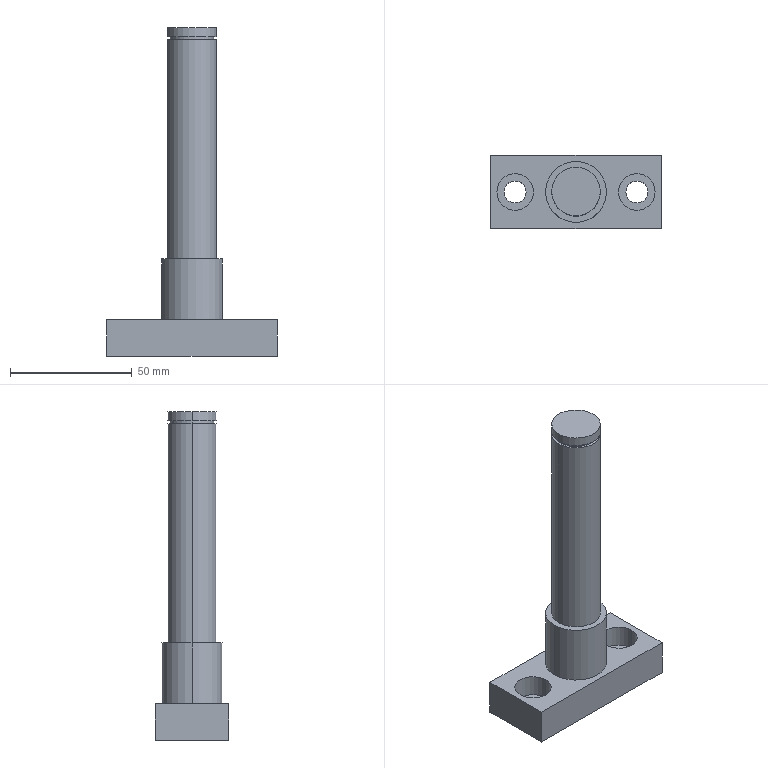Component | SolidWorks | -SmallRollerAssembly-1_-SmallPulleyBearingHousing-1 | 1 solid | 28 faces | box 70 x 30 x 135 mm | volume 69601 mm3 | cylinder 16 | plane 12 | commonest cylinder face diameters 15 x4 9 x4 20 x4 18 x2 25 x2
build123d program:
from build123d import *

# Parameters (mm, degrees)
SKETCH1_W                                           = 70
SKETCH1_H                                           = 30
BOSS_EXTRUDE1_DEPTH                                 = 15
SKETCH2_R                                           = 12.5
BOSS_EXTRUDE2_DEPTH                                 = 25
SKETCH3_R                                           = 10
BOSS_EXTRUDE3_DEPTH                                 = 95
SKETCH4_R                                           = 10
SKETCH4_R_2                                         = 9
CUT_EXTRUDE1_DEPTH                                  = 1.2
CYLINDRICAL_COUNTERSUNK_HOLE_FOR_M8_HEX_D           = 9
CYLINDRICAL_COUNTERSUNK_HOLE_FOR_M8_HEX_CBORE_D     = 15
CYLINDRICAL_COUNTERSUNK_HOLE_FOR_M8_HEX_CBORE_DEPTH = 9


with BuildPart() as part:
    # Sketch1 → Boss-Extrude1 (new body)
    with BuildSketch(Plane.XY):
        Rectangle(SKETCH1_W, SKETCH1_H)
    extrude(amount=BOSS_EXTRUDE1_DEPTH)

    # Sketch2 → Boss-Extrude2 (add)
    with BuildSketch(Plane.XY.offset(15)):
        Circle(SKETCH2_R)
    extrude(amount=BOSS_EXTRUDE2_DEPTH)

    # Sketch3 → Boss-Extrude3 (add)
    with BuildSketch(Plane.XY.offset(40)):
        Circle(SKETCH3_R)
    extrude(amount=BOSS_EXTRUDE3_DEPTH)

    # Sketch4 → Cut-Extrude1 (cut)
    with BuildSketch(Plane.XY.offset(130)):
        Circle(SKETCH4_R)
        Circle(SKETCH4_R_2, mode=Mode.SUBTRACT)
    extrude(amount=CUT_EXTRUDE1_DEPTH, mode=Mode.SUBTRACT)

    # Cylindrical Countersunk Hole for M8 Hex (through all)
    with Locations(Plane(origin=(0, 0, 15), x_dir=(-1, 0, 0), z_dir=(0, 0, 1))):
        with Locations((-25, 0), (25, 0)):
            CounterBoreHole(CYLINDRICAL_COUNTERSUNK_HOLE_FOR_M8_HEX_D / 2, CYLINDRICAL_COUNTERSUNK_HOLE_FOR_M8_HEX_CBORE_D / 2, CYLINDRICAL_COUNTERSUNK_HOLE_FOR_M8_HEX_CBORE_DEPTH)


solid = part.part

# Placed as in the assembly
solid = solid.moved(Location((-45, 1121, 5), (0, 0, 0)))
STEP:
#1=COLOUR_RGB('',0.7922,0.8196,0.9333);
#2=FILL_AREA_STYLE_COLOUR('',#1);
#3=FILL_AREA_STYLE('',(#2));
#4=SURFACE_STYLE_FILL_AREA(#3);
#5=SURFACE_SIDE_STYLE('',(#4));
#6=SURFACE_STYLE_USAGE(.BOTH.,#5);
#7=PRESENTATION_STYLE_ASSIGNMENT((#6));
#8=CARTESIAN_POINT('',(-1.083,44.134,0.4331));
#9=VERTEX_POINT('',#8);
#10=CARTESIAN_POINT('',(-0.4921,44.134,0.4331));
#11=VERTEX_POINT('',#10);
#12=CARTESIAN_POINT('',(-0.7874,44.134,0.4331));
#13=DIRECTION('',(0.,0.,1.));
#14=DIRECTION('',(1.,0.,0.));
#15=AXIS2_PLACEMENT_3D('',#12,#13,#14);
#16=CIRCLE('',#15,0.2953);
#17=EDGE_CURVE('',#9,#11,#16,.T.);
#18=ORIENTED_EDGE('',*,*,#17,.F.);
#19=CARTESIAN_POINT('',(-1.083,44.134,0.7874));
#20=VERTEX_POINT('',#19);
#21=CARTESIAN_POINT('',(-1.083,44.134,0.7874));
#22=DIRECTION('',(0.,0.,1.));
#23=VECTOR('',#22,39.37);
#24=LINE('',#21,#23);
#25=EDGE_CURVE('',#9,#20,#24,.T.);
#26=ORIENTED_EDGE('',*,*,#25,.T.);
#27=CARTESIAN_POINT('',(-0.4921,44.134,0.7874));
#28=VERTEX_POINT('',#27);
#29=CARTESIAN_POINT('',(-0.7874,44.134,0.7874));
#30=DIRECTION('',(0.,0.,1.));
#31=DIRECTION('',(1.,0.,0.));
#32=AXIS2_PLACEMENT_3D('',#29,#30,#31);
#33=CIRCLE('',#32,0.2953);
#34=EDGE_CURVE('',#20,#28,#33,.T.);
#35=ORIENTED_EDGE('',*,*,#34,.T.);
#36=CARTESIAN_POINT('',(-0.4921,44.134,0.7874));
#37=DIRECTION('',(0.,0.,1.));
#38=VECTOR('',#37,39.37);
#39=LINE('',#36,#38);
#40=EDGE_CURVE('',#11,#28,#39,.T.);
#41=ORIENTED_EDGE('',*,*,#40,.F.);
#42=EDGE_LOOP('',(#18,#26,#35,#41));
#43=FACE_OUTER_BOUND('',#42,.T.);
#44=CARTESIAN_POINT('',(-0.7874,44.134,0.7874));
#45=DIRECTION('',(0.,0.,1.));
#46=DIRECTION('',(1.,0.,0.));
#47=AXIS2_PLACEMENT_3D('',#44,#45,#46);
#48=CYLINDRICAL_SURFACE('',#47,0.2953);
#49=ADVANCED_FACE('',(#43),#48,.F.);
#50=CARTESIAN_POINT('',(-0.9646,44.134,0.1969));
#51=VERTEX_POINT('',#50);
#52=CARTESIAN_POINT('',(-0.6102,44.134,0.1969));
#53=VERTEX_POINT('',#52);
#54=CARTESIAN_POINT('',(-0.7874,44.134,0.1969));
#55=DIRECTION('',(0.,0.,1.));
#56=DIRECTION('',(1.,0.,0.));
#57=AXIS2_PLACEMENT_3D('',#54,#55,#56);
#58=CIRCLE('',#57,0.1772);
#59=EDGE_CURVE('',#51,#53,#58,.T.);
#60=ORIENTED_EDGE('',*,*,#59,.F.);
#61=CARTESIAN_POINT('',(-0.9646,44.134,0.4331));
#62=VERTEX_POINT('',#61);
#63=CARTESIAN_POINT('',(-0.9646,44.134,0.7874));
#64=DIRECTION('',(0.,0.,1.));
#65=VECTOR('',#64,39.37);
#66=LINE('',#63,#65);
#67=EDGE_CURVE('',#51,#62,#66,.T.);
#68=ORIENTED_EDGE('',*,*,#67,.T.);
#69=CARTESIAN_POINT('',(-0.6102,44.134,0.4331));
#70=VERTEX_POINT('',#69);
#71=CARTESIAN_POINT('',(-0.7874,44.134,0.4331));
#72=DIRECTION('',(0.,0.,1.));
#73=DIRECTION('',(1.,0.,0.));
#74=AXIS2_PLACEMENT_3D('',#71,#72,#73);
#75=CIRCLE('',#74,0.1772);
#76=EDGE_CURVE('',#62,#70,#75,.T.);
#77=ORIENTED_EDGE('',*,*,#76,.T.);
#78=CARTESIAN_POINT('',(-0.6102,44.134,0.7874));
#79=DIRECTION('',(0.,0.,1.));
#80=VECTOR('',#79,39.37);
#81=LINE('',#78,#80);
#82=EDGE_CURVE('',#53,#70,#81,.T.);
#83=ORIENTED_EDGE('',*,*,#82,.F.);
#84=EDGE_LOOP('',(#60,#68,#77,#83));
#85=FACE_OUTER_BOUND('',#84,.T.);
#86=CARTESIAN_POINT('',(-0.7874,44.134,0.7874));
#87=DIRECTION('',(0.,0.,1.));
#88=DIRECTION('',(1.,0.,0.));
#89=AXIS2_PLACEMENT_3D('',#86,#87,#88);
#90=CYLINDRICAL_SURFACE('',#89,0.1772);
#91=ADVANCED_FACE('',(#85),#90,.F.);
#92=CARTESIAN_POINT('',(-3.051,44.134,0.4331));
#93=VERTEX_POINT('',#92);
#94=CARTESIAN_POINT('',(-2.461,44.134,0.4331));
#95=VERTEX_POINT('',#94);
#96=CARTESIAN_POINT('',(-2.756,44.134,0.4331));
#97=DIRECTION('',(0.,0.,1.));
#98=DIRECTION('',(1.,0.,0.));
#99=AXIS2_PLACEMENT_3D('',#96,#97,#98);
#100=CIRCLE('',#99,0.2953);
#101=EDGE_CURVE('',#93,#95,#100,.T.);
#102=ORIENTED_EDGE('',*,*,#101,.F.);
#103=CARTESIAN_POINT('',(-3.051,44.134,0.7874));
#104=VERTEX_POINT('',#103);
#105=CARTESIAN_POINT('',(-3.051,44.134,0.7874));
#106=DIRECTION('',(0.,0.,1.));
#107=VECTOR('',#106,39.37);
#108=LINE('',#105,#107);
#109=EDGE_CURVE('',#93,#104,#108,.T.);
#110=ORIENTED_EDGE('',*,*,#109,.T.);
#111=CARTESIAN_POINT('',(-2.461,44.134,0.7874));
#112=VERTEX_POINT('',#111);
#113=CARTESIAN_POINT('',(-2.756,44.134,0.7874));
#114=DIRECTION('',(0.,0.,1.));
#115=DIRECTION('',(1.,0.,0.));
#116=AXIS2_PLACEMENT_3D('',#113,#114,#115);
#117=CIRCLE('',#116,0.2953);
#118=EDGE_CURVE('',#104,#112,#117,.T.);
#119=ORIENTED_EDGE('',*,*,#118,.T.);
#120=CARTESIAN_POINT('',(-2.461,44.134,0.7874));
#121=DIRECTION('',(0.,0.,1.));
#122=VECTOR('',#121,39.37);
#123=LINE('',#120,#122);
#124=EDGE_CURVE('',#95,#112,#123,.T.);
#125=ORIENTED_EDGE('',*,*,#124,.F.);
#126=EDGE_LOOP('',(#102,#110,#119,#125));
#127=FACE_OUTER_BOUND('',#126,.T.);
#128=CARTESIAN_POINT('',(-2.756,44.134,0.7874));
#129=DIRECTION('',(0.,0.,1.));
#130=DIRECTION('',(1.,0.,0.));
#131=AXIS2_PLACEMENT_3D('',#128,#129,#130);
#132=CYLINDRICAL_SURFACE('',#131,0.2953);
#133=ADVANCED_FACE('',(#127),#132,.F.);
#134=CARTESIAN_POINT('',(-2.933,44.134,0.1969));
#135=VERTEX_POINT('',#134);
#136=CARTESIAN_POINT('',(-2.579,44.134,0.1969));
#137=VERTEX_POINT('',#136);
#138=CARTESIAN_POINT('',(-2.756,44.134,0.1969));
#139=DIRECTION('',(0.,0.,1.));
#140=DIRECTION('',(1.,0.,0.));
#141=AXIS2_PLACEMENT_3D('',#138,#139,#140);
#142=CIRCLE('',#141,0.1772);
#143=EDGE_CURVE('',#135,#137,#142,.T.);
#144=ORIENTED_EDGE('',*,*,#143,.F.);
#145=CARTESIAN_POINT('',(-2.933,44.134,0.4331));
#146=VERTEX_POINT('',#145);
#147=CARTESIAN_POINT('',(-2.933,44.134,0.7874));
#148=DIRECTION('',(0.,0.,1.));
#149=VECTOR('',#148,39.37);
#150=LINE('',#147,#149);
#151=EDGE_CURVE('',#135,#146,#150,.T.);
#152=ORIENTED_EDGE('',*,*,#151,.T.);
#153=CARTESIAN_POINT('',(-2.579,44.134,0.4331));
#154=VERTEX_POINT('',#153);
#155=CARTESIAN_POINT('',(-2.756,44.134,0.4331));
#156=DIRECTION('',(0.,0.,1.));
#157=DIRECTION('',(1.,0.,0.));
#158=AXIS2_PLACEMENT_3D('',#155,#156,#157);
#159=CIRCLE('',#158,0.1772);
#160=EDGE_CURVE('',#146,#154,#159,.T.);
#161=ORIENTED_EDGE('',*,*,#160,.T.);
#162=CARTESIAN_POINT('',(-2.579,44.134,0.7874));
#163=DIRECTION('',(0.,0.,1.));
#164=VECTOR('',#163,39.37);
#165=LINE('',#162,#164);
#166=EDGE_CURVE('',#137,#154,#165,.T.);
#167=ORIENTED_EDGE('',*,*,#166,.F.);
#168=EDGE_LOOP('',(#144,#152,#161,#167));
#169=FACE_OUTER_BOUND('',#168,.T.);
#170=CARTESIAN_POINT('',(-2.756,44.134,0.7874));
#171=DIRECTION('',(0.,0.,1.));
#172=DIRECTION('',(1.,0.,0.));
#173=AXIS2_PLACEMENT_3D('',#170,#171,#172);
#174=CYLINDRICAL_SURFACE('',#173,0.1772);
#175=ADVANCED_FACE('',(#169),#174,.F.);
#176=CARTESIAN_POINT('',(-1.378,44.134,5.512));
#177=VERTEX_POINT('',#176);
#178=CARTESIAN_POINT('',(-2.165,44.134,5.512));
#179=VERTEX_POINT('',#178);
#180=CARTESIAN_POINT('',(-1.772,44.134,5.512));
#181=DIRECTION('',(0.,0.,1.));
#182=DIRECTION('',(1.,0.,0.));
#183=AXIS2_PLACEMENT_3D('',#180,#181,#182);
#184=CIRCLE('',#183,0.3937);
#185=EDGE_CURVE('',#177,#179,#184,.T.);
#186=ORIENTED_EDGE('',*,*,#185,.F.);
#187=CARTESIAN_POINT('',(-1.378,44.134,5.362));
#188=VERTEX_POINT('',#187);
#189=CARTESIAN_POINT('',(-1.378,44.134,5.512));
#190=DIRECTION('',(0.,0.,-1.));
#191=VECTOR('',#190,39.37);
#192=LINE('',#189,#191);
#193=EDGE_CURVE('',#177,#188,#192,.T.);
#194=ORIENTED_EDGE('',*,*,#193,.T.);
#195=CARTESIAN_POINT('',(-2.165,44.134,5.362));
#196=VERTEX_POINT('',#195);
#197=CARTESIAN_POINT('',(-1.772,44.134,5.362));
#198=DIRECTION('',(0.,0.,1.));
#199=DIRECTION('',(1.,0.,0.));
#200=AXIS2_PLACEMENT_3D('',#197,#198,#199);
#201=CIRCLE('',#200,0.3937);
#202=EDGE_CURVE('',#188,#196,#201,.T.);
#203=ORIENTED_EDGE('',*,*,#202,.T.);
#204=CARTESIAN_POINT('',(-2.165,44.134,5.512));
#205=DIRECTION('',(0.,0.,-1.));
#206=VECTOR('',#205,39.37);
#207=LINE('',#204,#206);
#208=EDGE_CURVE('',#179,#196,#207,.T.);
#209=ORIENTED_EDGE('',*,*,#208,.F.);
#210=EDGE_LOOP('',(#186,#194,#203,#209));
#211=FACE_OUTER_BOUND('',#210,.T.);
#212=CARTESIAN_POINT('',(-1.772,44.134,5.512));
#213=DIRECTION('',(0.,0.,-1.));
#214=DIRECTION('',(-1.,0.,0.));
#215=AXIS2_PLACEMENT_3D('',#212,#213,#214);
#216=CYLINDRICAL_SURFACE('',#215,0.3937);
#217=ADVANCED_FACE('',(#211),#216,.T.);
#218=CARTESIAN_POINT('',(-1.417,44.134,5.362));
#219=VERTEX_POINT('',#218);
#220=CARTESIAN_POINT('',(-2.126,44.134,5.362));
#221=VERTEX_POINT('',#220);
#222=CARTESIAN_POINT('',(-1.772,44.134,5.362));
#223=DIRECTION('',(0.,0.,1.));
#224=DIRECTION('',(1.,0.,0.));
#225=AXIS2_PLACEMENT_3D('',#222,#223,#224);
#226=CIRCLE('',#225,0.3543);
#227=EDGE_CURVE('',#219,#221,#226,.T.);
#228=ORIENTED_EDGE('',*,*,#227,.F.);
#229=CARTESIAN_POINT('',(-1.417,44.134,5.315));
#230=VERTEX_POINT('',#229);
#231=CARTESIAN_POINT('',(-1.417,44.134,5.362));
#232=DIRECTION('',(0.,0.,-1.));
#233=VECTOR('',#232,39.37);
#234=LINE('',#231,#233);
#235=EDGE_CURVE('',#219,#230,#234,.T.);
#236=ORIENTED_EDGE('',*,*,#235,.T.);
#237=CARTESIAN_POINT('',(-2.126,44.134,5.315));
#238=VERTEX_POINT('',#237);
#239=CARTESIAN_POINT('',(-1.772,44.134,5.315));
#240=DIRECTION('',(0.,0.,1.));
#241=DIRECTION('',(1.,0.,0.));
#242=AXIS2_PLACEMENT_3D('',#239,#240,#241);
#243=CIRCLE('',#242,0.3543);
#244=EDGE_CURVE('',#230,#238,#243,.T.);
#245=ORIENTED_EDGE('',*,*,#244,.T.);
#246=CARTESIAN_POINT('',(-2.126,44.134,5.362));
#247=DIRECTION('',(0.,0.,-1.));
#248=VECTOR('',#247,39.37);
#249=LINE('',#246,#248);
#250=EDGE_CURVE('',#221,#238,#249,.T.);
#251=ORIENTED_EDGE('',*,*,#250,.F.);
#252=EDGE_LOOP('',(#228,#236,#245,#251));
#253=FACE_OUTER_BOUND('',#252,.T.);
#254=CARTESIAN_POINT('',(-1.772,44.134,5.362));
#255=DIRECTION('',(0.,0.,-1.));
#256=DIRECTION('',(-1.,0.,0.));
#257=AXIS2_PLACEMENT_3D('',#254,#255,#256);
#258=CYLINDRICAL_SURFACE('',#257,0.3543);
#259=ADVANCED_FACE('',(#253),#258,.T.);
#260=CARTESIAN_POINT('',(-1.28,44.134,1.772));
#261=VERTEX_POINT('',#260);
#262=CARTESIAN_POINT('',(-2.264,44.134,1.772));
#263=VERTEX_POINT('',#262);
#264=CARTESIAN_POINT('',(-1.772,44.134,1.772));
#265=DIRECTION('',(0.,0.,1.));
#266=DIRECTION('',(1.,0.,0.));
#267=AXIS2_PLACEMENT_3D('',#264,#265,#266);
#268=CIRCLE('',#267,0.4921);
#269=EDGE_CURVE('',#261,#263,#268,.T.);
#270=ORIENTED_EDGE('',*,*,#269,.F.);
#271=CARTESIAN_POINT('',(-1.28,44.134,0.7874));
#272=VERTEX_POINT('',#271);
#273=CARTESIAN_POINT('',(-1.28,44.134,1.772));
#274=DIRECTION('',(0.,0.,-1.));
#275=VECTOR('',#274,39.37);
#276=LINE('',#273,#275);
#277=EDGE_CURVE('',#261,#272,#276,.T.);
#278=ORIENTED_EDGE('',*,*,#277,.T.);
#279=CARTESIAN_POINT('',(-2.264,44.134,0.7874));
#280=VERTEX_POINT('',#279);
#281=CARTESIAN_POINT('',(-1.772,44.134,0.7874));
#282=DIRECTION('',(0.,0.,1.));
#283=DIRECTION('',(1.,0.,0.));
#284=AXIS2_PLACEMENT_3D('',#281,#282,#283);
#285=CIRCLE('',#284,0.4921);
#286=EDGE_CURVE('',#272,#280,#285,.T.);
#287=ORIENTED_EDGE('',*,*,#286,.T.);
#288=CARTESIAN_POINT('',(-2.264,44.134,1.772));
#289=DIRECTION('',(0.,0.,-1.));
#290=VECTOR('',#289,39.37);
#291=LINE('',#288,#290);
#292=EDGE_CURVE('',#263,#280,#291,.T.);
#293=ORIENTED_EDGE('',*,*,#292,.F.);
#294=EDGE_LOOP('',(#270,#278,#287,#293));
#295=FACE_OUTER_BOUND('',#294,.T.);
#296=CARTESIAN_POINT('',(-1.772,44.134,1.772));
#297=DIRECTION('',(0.,0.,-1.));
#298=DIRECTION('',(-1.,0.,0.));
#299=AXIS2_PLACEMENT_3D('',#296,#297,#298);
#300=CYLINDRICAL_SURFACE('',#299,0.4921);
#301=ADVANCED_FACE('',(#295),#300,.T.);
#302=CARTESIAN_POINT('',(-1.378,44.134,5.315));
#303=VERTEX_POINT('',#302);
#304=CARTESIAN_POINT('',(-2.165,44.134,5.315));
#305=VERTEX_POINT('',#304);
#306=CARTESIAN_POINT('',(-1.772,44.134,5.315));
#307=DIRECTION('',(0.,0.,1.));
#308=DIRECTION('',(1.,0.,0.));
#309=AXIS2_PLACEMENT_3D('',#306,#307,#308);
#310=CIRCLE('',#309,0.3937);
#311=EDGE_CURVE('',#303,#305,#310,.T.);
#312=ORIENTED_EDGE('',*,*,#311,.F.);
#313=CARTESIAN_POINT('',(-1.378,44.134,1.772));
#314=VERTEX_POINT('',#313);
#315=CARTESIAN_POINT('',(-1.378,44.134,5.512));
#316=DIRECTION('',(0.,0.,-1.));
#317=VECTOR('',#316,39.37);
#318=LINE('',#315,#317);
#319=EDGE_CURVE('',#303,#314,#318,.T.);
#320=ORIENTED_EDGE('',*,*,#319,.T.);
#321=CARTESIAN_POINT('',(-2.165,44.134,1.772));
#322=VERTEX_POINT('',#321);
#323=CARTESIAN_POINT('',(-1.772,44.134,1.772));
#324=DIRECTION('',(0.,0.,1.));
#325=DIRECTION('',(1.,0.,0.));
#326=AXIS2_PLACEMENT_3D('',#323,#324,#325);
#327=CIRCLE('',#326,0.3937);
#328=EDGE_CURVE('',#314,#322,#327,.T.);
#329=ORIENTED_EDGE('',*,*,#328,.T.);
#330=CARTESIAN_POINT('',(-2.165,44.134,5.512));
#331=DIRECTION('',(0.,0.,-1.));
#332=VECTOR('',#331,39.37);
#333=LINE('',#330,#332);
#334=EDGE_CURVE('',#305,#322,#333,.T.);
#335=ORIENTED_EDGE('',*,*,#334,.F.);
#336=EDGE_LOOP('',(#312,#320,#329,#335));
#337=FACE_OUTER_BOUND('',#336,.T.);
#338=CARTESIAN_POINT('',(-1.772,44.134,5.512));
#339=DIRECTION('',(0.,0.,-1.));
#340=DIRECTION('',(-1.,0.,0.));
#341=AXIS2_PLACEMENT_3D('',#338,#339,#340);
#342=CYLINDRICAL_SURFACE('',#341,0.3937);
#343=ADVANCED_FACE('',(#337),#342,.T.);
#344=ORIENTED_EDGE('',*,*,#319,.F.);
#345=CARTESIAN_POINT('',(-1.772,44.134,5.315));
#346=DIRECTION('',(0.,0.,1.));
#347=DIRECTION('',(1.,0.,0.));
#348=AXIS2_PLACEMENT_3D('',#345,#346,#347);
#349=CIRCLE('',#348,0.3937);
#350=EDGE_CURVE('',#305,#303,#349,.T.);
#351=ORIENTED_EDGE('',*,*,#350,.F.);
#352=ORIENTED_EDGE('',*,*,#334,.T.);
#353=CARTESIAN_POINT('',(-1.772,44.134,1.772));
#354=DIRECTION('',(0.,0.,1.));
#355=DIRECTION('',(1.,0.,0.));
#356=AXIS2_PLACEMENT_3D('',#353,#354,#355);
#357=CIRCLE('',#356,0.3937);
#358=EDGE_CURVE('',#322,#314,#357,.T.);
#359=ORIENTED_EDGE('',*,*,#358,.T.);
#360=EDGE_LOOP('',(#344,#351,#352,#359));
#361=FACE_OUTER_BOUND('',#360,.T.);
#362=CARTESIAN_POINT('',(-1.772,44.134,5.512));
#363=DIRECTION('',(0.,0.,-1.));
#364=DIRECTION('',(-1.,0.,0.));
#365=AXIS2_PLACEMENT_3D('',#362,#363,#364);
#366=CYLINDRICAL_SURFACE('',#365,0.3937);
#367=ADVANCED_FACE('',(#361),#366,.T.);
#368=CARTESIAN_POINT('',(-1.772,44.134,1.772));
#369=DIRECTION('',(0.,0.,1.));
#370=DIRECTION('',(1.,0.,0.));
#371=AXIS2_PLACEMENT_3D('',#368,#369,#370);
#372=CIRCLE('',#371,0.4921);
#373=EDGE_CURVE('',#263,#261,#372,.T.);
#374=ORIENTED_EDGE('',*,*,#373,.T.);
#375=ORIENTED_EDGE('',*,*,#269,.T.);
#376=EDGE_LOOP('',(#374,#375));
#377=FACE_OUTER_BOUND('',#376,.T.);
#378=ORIENTED_EDGE('',*,*,#358,.F.);
#379=ORIENTED_EDGE('',*,*,#328,.F.);
#380=EDGE_LOOP('',(#378,#379));
#381=FACE_BOUND('',#380,.T.);
#382=CARTESIAN_POINT('',(-1.772,44.134,1.772));
#383=DIRECTION('',(0.,0.,1.));
#384=DIRECTION('',(1.,0.,0.));
#385=AXIS2_PLACEMENT_3D('',#382,#383,#384);
#386=PLANE('',#385);
#387=ADVANCED_FACE('',(#377,#381),#386,.T.);
#388=CARTESIAN_POINT('',(-0.7874,44.134,0.7874));
#389=DIRECTION('',(0.,0.,1.));
#390=DIRECTION('',(1.,0.,0.));
#391=AXIS2_PLACEMENT_3D('',#388,#389,#390);
#392=CIRCLE('',#391,0.2953);
#393=EDGE_CURVE('',#28,#20,#392,.T.);
#394=ORIENTED_EDGE('',*,*,#393,.F.);
#395=ORIENTED_EDGE('',*,*,#34,.F.);
#396=EDGE_LOOP('',(#394,#395));
#397=FACE_BOUND('',#396,.T.);
#398=CARTESIAN_POINT('',(-2.756,44.134,0.7874));
#399=DIRECTION('',(0.,0.,1.));
#400=DIRECTION('',(1.,0.,0.));
#401=AXIS2_PLACEMENT_3D('',#398,#399,#400);
#402=CIRCLE('',#401,0.2953);
#403=EDGE_CURVE('',#112,#104,#402,.T.);
#404=ORIENTED_EDGE('',*,*,#403,.F.);
#405=ORIENTED_EDGE('',*,*,#118,.F.);
#406=EDGE_LOOP('',(#404,#405));
#407=FACE_BOUND('',#406,.T.);
#408=CARTESIAN_POINT('',(-3.15,44.724,0.7874));
#409=VERTEX_POINT('',#408);
#410=CARTESIAN_POINT('',(-3.15,43.543,0.7874));
#411=VERTEX_POINT('',#410);
#412=CARTESIAN_POINT('',(-3.15,43.543,0.7874));
#413=DIRECTION('',(0.,-1.,0.));
#414=VECTOR('',#413,39.37);
#415=LINE('',#412,#414);
#416=EDGE_CURVE('',#409,#411,#415,.T.);
#417=ORIENTED_EDGE('',*,*,#416,.T.);
#418=CARTESIAN_POINT('',(-0.3937,43.543,0.7874));
#419=VERTEX_POINT('',#418);
#420=CARTESIAN_POINT('',(-0.3937,43.543,0.7874));
#421=DIRECTION('',(1.,0.,0.));
#422=VECTOR('',#421,39.37);
#423=LINE('',#420,#422);
#424=EDGE_CURVE('',#411,#419,#423,.T.);
#425=ORIENTED_EDGE('',*,*,#424,.T.);
#426=CARTESIAN_POINT('',(-0.3937,44.724,0.7874));
#427=VERTEX_POINT('',#426);
#428=CARTESIAN_POINT('',(-0.3937,43.543,0.7874));
#429=DIRECTION('',(0.,1.,0.));
#430=VECTOR('',#429,39.37);
#431=LINE('',#428,#430);
#432=EDGE_CURVE('',#419,#427,#431,.T.);
#433=ORIENTED_EDGE('',*,*,#432,.T.);
#434=CARTESIAN_POINT('',(-0.3937,44.724,0.7874));
#435=DIRECTION('',(-1.,-0.,0.));
#436=VECTOR('',#435,39.37);
#437=LINE('',#434,#436);
#438=EDGE_CURVE('',#427,#409,#437,.T.);
#439=ORIENTED_EDGE('',*,*,#438,.T.);
#440=EDGE_LOOP('',(#417,#425,#433,#439));
#441=FACE_OUTER_BOUND('',#440,.T.);
#442=CARTESIAN_POINT('',(-1.772,44.134,0.7874));
#443=DIRECTION('',(0.,0.,1.));
#444=DIRECTION('',(1.,0.,0.));
#445=AXIS2_PLACEMENT_3D('',#442,#443,#444);
#446=CIRCLE('',#445,0.4921);
#447=EDGE_CURVE('',#280,#272,#446,.T.);
#448=ORIENTED_EDGE('',*,*,#447,.F.);
#449=ORIENTED_EDGE('',*,*,#286,.F.);
#450=EDGE_LOOP('',(#448,#449));
#451=FACE_BOUND('',#450,.T.);
#452=CARTESIAN_POINT('',(-1.772,44.134,0.7874));
#453=DIRECTION('',(0.,0.,1.));
#454=DIRECTION('',(1.,0.,0.));
#455=AXIS2_PLACEMENT_3D('',#452,#453,#454);
#456=PLANE('',#455);
#457=ADVANCED_FACE('',(#397,#407,#441,#451),#456,.T.);
#458=CARTESIAN_POINT('',(-3.15,44.724,0.1969));
#459=VERTEX_POINT('',#458);
#460=CARTESIAN_POINT('',(-3.15,43.543,0.1969));
#461=VERTEX_POINT('',#460);
#462=CARTESIAN_POINT('',(-3.15,43.543,0.1969));
#463=DIRECTION('',(0.,-1.,0.));
#464=VECTOR('',#463,39.37);
#465=LINE('',#462,#464);
#466=EDGE_CURVE('',#459,#461,#465,.T.);
#467=ORIENTED_EDGE('',*,*,#466,.T.);
#468=CARTESIAN_POINT('',(-3.15,43.543,0.7874));
#469=DIRECTION('',(0.,0.,-1.));
#470=VECTOR('',#469,39.37);
#471=LINE('',#468,#470);
#472=EDGE_CURVE('',#411,#461,#471,.T.);
#473=ORIENTED_EDGE('',*,*,#472,.F.);
#474=ORIENTED_EDGE('',*,*,#416,.F.);
#475=CARTESIAN_POINT('',(-3.15,44.724,0.7874));
#476=DIRECTION('',(0.,0.,-1.));
#477=VECTOR('',#476,39.37);
#478=LINE('',#475,#477);
#479=EDGE_CURVE('',#409,#459,#478,.T.);
#480=ORIENTED_EDGE('',*,*,#479,.T.);
#481=EDGE_LOOP('',(#467,#473,#474,#480));
#482=FACE_OUTER_BOUND('',#481,.T.);
#483=CARTESIAN_POINT('',(-3.15,43.543,0.7874));
#484=DIRECTION('',(1.,0.,0.));
#485=DIRECTION('',(0.,0.,-1.));
#486=AXIS2_PLACEMENT_3D('',#483,#484,#485);
#487=PLANE('',#486);
#488=ADVANCED_FACE('',(#482),#487,.F.);
#489=CARTESIAN_POINT('',(-0.3937,43.543,0.1969));
#490=VERTEX_POINT('',#489);
#491=CARTESIAN_POINT('',(-0.3937,43.543,0.1969));
#492=DIRECTION('',(1.,0.,0.));
#493=VECTOR('',#492,39.37);
#494=LINE('',#491,#493);
#495=EDGE_CURVE('',#461,#490,#494,.T.);
#496=ORIENTED_EDGE('',*,*,#495,.T.);
#497=CARTESIAN_POINT('',(-0.3937,43.543,0.7874));
#498=DIRECTION('',(0.,0.,-1.));
#499=VECTOR('',#498,39.37);
#500=LINE('',#497,#499);
#501=EDGE_CURVE('',#419,#490,#500,.T.);
#502=ORIENTED_EDGE('',*,*,#501,.F.);
#503=ORIENTED_EDGE('',*,*,#424,.F.);
#504=ORIENTED_EDGE('',*,*,#472,.T.);
#505=EDGE_LOOP('',(#496,#502,#503,#504));
#506=FACE_OUTER_BOUND('',#505,.T.);
#507=CARTESIAN_POINT('',(-0.3937,43.543,0.7874));
#508=DIRECTION('',(-0.,1.,0.));
#509=DIRECTION('',(-1.,-0.,0.));
#510=AXIS2_PLACEMENT_3D('',#507,#508,#509);
#511=PLANE('',#510);
#512=ADVANCED_FACE('',(#506),#511,.F.);
#513=CARTESIAN_POINT('',(-0.3937,44.724,0.1969));
#514=VERTEX_POINT('',#513);
#515=CARTESIAN_POINT('',(-0.3937,43.543,0.1969));
#516=DIRECTION('',(0.,1.,0.));
#517=VECTOR('',#516,39.37);
#518=LINE('',#515,#517);
#519=EDGE_CURVE('',#490,#514,#518,.T.);
#520=ORIENTED_EDGE('',*,*,#519,.T.);
#521=CARTESIAN_POINT('',(-0.3937,44.724,0.7874));
#522=DIRECTION('',(0.,0.,-1.));
#523=VECTOR('',#522,39.37);
#524=LINE('',#521,#523);
#525=EDGE_CURVE('',#427,#514,#524,.T.);
#526=ORIENTED_EDGE('',*,*,#525,.F.);
#527=ORIENTED_EDGE('',*,*,#432,.F.);
#528=ORIENTED_EDGE('',*,*,#501,.T.);
#529=EDGE_LOOP('',(#520,#526,#527,#528));
#530=FACE_OUTER_BOUND('',#529,.T.);
#531=CARTESIAN_POINT('',(-0.3937,43.543,0.7874));
#532=DIRECTION('',(-1.,0.,0.));
#533=DIRECTION('',(0.,0.,1.));
#534=AXIS2_PLACEMENT_3D('',#531,#532,#533);
#535=PLANE('',#534);
#536=ADVANCED_FACE('',(#530),#535,.F.);
#537=CARTESIAN_POINT('',(-0.3937,44.724,0.1969));
#538=DIRECTION('',(-1.,-0.,0.));
#539=VECTOR('',#538,39.37);
#540=LINE('',#537,#539);
#541=EDGE_CURVE('',#514,#459,#540,.T.);
#542=ORIENTED_EDGE('',*,*,#541,.T.);
#543=ORIENTED_EDGE('',*,*,#479,.F.);
#544=ORIENTED_EDGE('',*,*,#438,.F.);
#545=ORIENTED_EDGE('',*,*,#525,.T.);
#546=EDGE_LOOP('',(#542,#543,#544,#545));
#547=FACE_OUTER_BOUND('',#546,.T.);
#548=CARTESIAN_POINT('',(-0.3937,44.724,0.7874));
#549=DIRECTION('',(0.,-1.,0.));
#550=DIRECTION('',(1.,0.,0.));
#551=AXIS2_PLACEMENT_3D('',#548,#549,#550);
#552=PLANE('',#551);
#553=ADVANCED_FACE('',(#547),#552,.F.);
#554=CARTESIAN_POINT('',(-0.7874,44.134,0.1969));
#555=DIRECTION('',(0.,0.,1.));
#556=DIRECTION('',(1.,0.,0.));
#557=AXIS2_PLACEMENT_3D('',#554,#555,#556);
#558=CIRCLE('',#557,0.1772);
#559=EDGE_CURVE('',#53,#51,#558,.T.);
#560=ORIENTED_EDGE('',*,*,#559,.T.);
#561=ORIENTED_EDGE('',*,*,#59,.T.);
#562=EDGE_LOOP('',(#560,#561));
#563=FACE_BOUND('',#562,.T.);
#564=CARTESIAN_POINT('',(-2.756,44.134,0.1969));
#565=DIRECTION('',(0.,0.,1.));
#566=DIRECTION('',(1.,0.,0.));
#567=AXIS2_PLACEMENT_3D('',#564,#565,#566);
#568=CIRCLE('',#567,0.1772);
#569=EDGE_CURVE('',#137,#135,#568,.T.);
#570=ORIENTED_EDGE('',*,*,#569,.T.);
#571=ORIENTED_EDGE('',*,*,#143,.T.);
#572=EDGE_LOOP('',(#570,#571));
#573=FACE_BOUND('',#572,.T.);
#574=ORIENTED_EDGE('',*,*,#466,.F.);
#575=ORIENTED_EDGE('',*,*,#541,.F.);
#576=ORIENTED_EDGE('',*,*,#519,.F.);
#577=ORIENTED_EDGE('',*,*,#495,.F.);
#578=EDGE_LOOP('',(#574,#575,#576,#577));
#579=FACE_OUTER_BOUND('',#578,.T.);
#580=CARTESIAN_POINT('',(-1.772,44.134,0.1969));
#581=DIRECTION('',(0.,0.,1.));
#582=DIRECTION('',(1.,0.,0.));
#583=AXIS2_PLACEMENT_3D('',#580,#581,#582);
#584=PLANE('',#583);
#585=ADVANCED_FACE('',(#563,#573,#579),#584,.F.);
#586=ORIENTED_EDGE('',*,*,#277,.F.);
#587=ORIENTED_EDGE('',*,*,#373,.F.);
#588=ORIENTED_EDGE('',*,*,#292,.T.);
#589=ORIENTED_EDGE('',*,*,#447,.T.);
#590=EDGE_LOOP('',(#586,#587,#588,#589));
#591=FACE_OUTER_BOUND('',#590,.T.);
#592=CARTESIAN_POINT('',(-1.772,44.134,1.772));
#593=DIRECTION('',(0.,0.,-1.));
#594=DIRECTION('',(-1.,0.,0.));
#595=AXIS2_PLACEMENT_3D('',#592,#593,#594);
#596=CYLINDRICAL_SURFACE('',#595,0.4921);
#597=ADVANCED_FACE('',(#591),#596,.T.);
#598=CARTESIAN_POINT('',(-1.772,44.134,5.362));
#599=DIRECTION('',(0.,0.,1.));
#600=DIRECTION('',(1.,0.,0.));
#601=AXIS2_PLACEMENT_3D('',#598,#599,#600);
#602=CIRCLE('',#601,0.3937);
#603=EDGE_CURVE('',#196,#188,#602,.T.);
#604=ORIENTED_EDGE('',*,*,#603,.F.);
#605=ORIENTED_EDGE('',*,*,#202,.F.);
#606=EDGE_LOOP('',(#604,#605));
#607=FACE_OUTER_BOUND('',#606,.T.);
#608=CARTESIAN_POINT('',(-1.772,44.134,5.362));
#609=DIRECTION('',(0.,0.,1.));
#610=DIRECTION('',(1.,0.,0.));
#611=AXIS2_PLACEMENT_3D('',#608,#609,#610);
#612=CIRCLE('',#611,0.3543);
#613=EDGE_CURVE('',#221,#219,#612,.T.);
#614=ORIENTED_EDGE('',*,*,#613,.T.);
#615=ORIENTED_EDGE('',*,*,#227,.T.);
#616=EDGE_LOOP('',(#614,#615));
#617=FACE_BOUND('',#616,.T.);
#618=CARTESIAN_POINT('',(-1.772,44.134,5.362));
#619=DIRECTION('',(0.,0.,1.));
#620=DIRECTION('',(1.,0.,0.));
#621=AXIS2_PLACEMENT_3D('',#618,#619,#620);
#622=PLANE('',#621);
#623=ADVANCED_FACE('',(#607,#617),#622,.F.);
#624=ORIENTED_EDGE('',*,*,#350,.T.);
#625=ORIENTED_EDGE('',*,*,#311,.T.);
#626=EDGE_LOOP('',(#624,#625));
#627=FACE_OUTER_BOUND('',#626,.T.);
#628=CARTESIAN_POINT('',(-1.772,44.134,5.315));
#629=DIRECTION('',(0.,0.,1.));
#630=DIRECTION('',(1.,0.,0.));
#631=AXIS2_PLACEMENT_3D('',#628,#629,#630);
#632=CIRCLE('',#631,0.3543);
#633=EDGE_CURVE('',#238,#230,#632,.T.);
#634=ORIENTED_EDGE('',*,*,#633,.F.);
#635=ORIENTED_EDGE('',*,*,#244,.F.);
#636=EDGE_LOOP('',(#634,#635));
#637=FACE_BOUND('',#636,.T.);
#638=CARTESIAN_POINT('',(-1.772,44.134,5.315));
#639=DIRECTION('',(0.,0.,1.));
#640=DIRECTION('',(1.,0.,0.));
#641=AXIS2_PLACEMENT_3D('',#638,#639,#640);
#642=PLANE('',#641);
#643=ADVANCED_FACE('',(#627,#637),#642,.T.);
#644=ORIENTED_EDGE('',*,*,#235,.F.);
#645=ORIENTED_EDGE('',*,*,#613,.F.);
#646=ORIENTED_EDGE('',*,*,#250,.T.);
#647=ORIENTED_EDGE('',*,*,#633,.T.);
#648=EDGE_LOOP('',(#644,#645,#646,#647));
#649=FACE_OUTER_BOUND('',#648,.T.);
#650=CARTESIAN_POINT('',(-1.772,44.134,5.362));
#651=DIRECTION('',(0.,0.,-1.));
#652=DIRECTION('',(-1.,0.,0.));
#653=AXIS2_PLACEMENT_3D('',#650,#651,#652);
#654=CYLINDRICAL_SURFACE('',#653,0.3543);
#655=ADVANCED_FACE('',(#649),#654,.T.);
#656=CARTESIAN_POINT('',(-1.772,44.134,5.512));
#657=DIRECTION('',(0.,0.,1.));
#658=DIRECTION('',(1.,0.,0.));
#659=AXIS2_PLACEMENT_3D('',#656,#657,#658);
#660=CIRCLE('',#659,0.3937);
#661=EDGE_CURVE('',#179,#177,#660,.T.);
#662=ORIENTED_EDGE('',*,*,#661,.T.);
#663=ORIENTED_EDGE('',*,*,#185,.T.);
#664=EDGE_LOOP('',(#662,#663));
#665=FACE_OUTER_BOUND('',#664,.T.);
#666=CARTESIAN_POINT('',(-1.772,44.134,5.512));
#667=DIRECTION('',(0.,0.,1.));
#668=DIRECTION('',(1.,0.,0.));
#669=AXIS2_PLACEMENT_3D('',#666,#667,#668);
#670=PLANE('',#669);
#671=ADVANCED_FACE('',(#665),#670,.T.);
#672=ORIENTED_EDGE('',*,*,#193,.F.);
#673=ORIENTED_EDGE('',*,*,#661,.F.);
#674=ORIENTED_EDGE('',*,*,#208,.T.);
#675=ORIENTED_EDGE('',*,*,#603,.T.);
#676=EDGE_LOOP('',(#672,#673,#674,#675));
#677=FACE_OUTER_BOUND('',#676,.T.);
#678=CARTESIAN_POINT('',(-1.772,44.134,5.512));
#679=DIRECTION('',(0.,0.,-1.));
#680=DIRECTION('',(-1.,0.,0.));
#681=AXIS2_PLACEMENT_3D('',#678,#679,#680);
#682=CYLINDRICAL_SURFACE('',#681,0.3937);
#683=ADVANCED_FACE('',(#677),#682,.T.);
#684=ORIENTED_EDGE('',*,*,#151,.F.);
#685=ORIENTED_EDGE('',*,*,#569,.F.);
#686=ORIENTED_EDGE('',*,*,#166,.T.);
#687=CARTESIAN_POINT('',(-2.756,44.134,0.4331));
#688=DIRECTION('',(0.,0.,1.));
#689=DIRECTION('',(1.,0.,0.));
#690=AXIS2_PLACEMENT_3D('',#687,#688,#689);
#691=CIRCLE('',#690,0.1772);
#692=EDGE_CURVE('',#154,#146,#691,.T.);
#693=ORIENTED_EDGE('',*,*,#692,.T.);
#694=EDGE_LOOP('',(#684,#685,#686,#693));
#695=FACE_OUTER_BOUND('',#694,.T.);
#696=CARTESIAN_POINT('',(-2.756,44.134,0.7874));
#697=DIRECTION('',(0.,0.,1.));
#698=DIRECTION('',(1.,0.,0.));
#699=AXIS2_PLACEMENT_3D('',#696,#697,#698);
#700=CYLINDRICAL_SURFACE('',#699,0.1772);
#701=ADVANCED_FACE('',(#695),#700,.F.);
#702=ORIENTED_EDGE('',*,*,#692,.F.);
#703=ORIENTED_EDGE('',*,*,#160,.F.);
#704=EDGE_LOOP('',(#702,#703));
#705=FACE_BOUND('',#704,.T.);
#706=CARTESIAN_POINT('',(-2.756,44.134,0.4331));
#707=DIRECTION('',(0.,0.,1.));
#708=DIRECTION('',(1.,0.,0.));
#709=AXIS2_PLACEMENT_3D('',#706,#707,#708);
#710=CIRCLE('',#709,0.2953);
#711=EDGE_CURVE('',#95,#93,#710,.T.);
#712=ORIENTED_EDGE('',*,*,#711,.T.);
#713=ORIENTED_EDGE('',*,*,#101,.T.);
#714=EDGE_LOOP('',(#712,#713));
#715=FACE_OUTER_BOUND('',#714,.T.);
#716=CARTESIAN_POINT('',(-2.579,44.134,0.4331));
#717=DIRECTION('',(0.,0.,-1.));
#718=DIRECTION('',(-1.,0.,0.));
#719=AXIS2_PLACEMENT_3D('',#716,#717,#718);
#720=PLANE('',#719);
#721=ADVANCED_FACE('',(#705,#715),#720,.F.);
#722=ORIENTED_EDGE('',*,*,#109,.F.);
#723=ORIENTED_EDGE('',*,*,#711,.F.);
#724=ORIENTED_EDGE('',*,*,#124,.T.);
#725=ORIENTED_EDGE('',*,*,#403,.T.);
#726=EDGE_LOOP('',(#722,#723,#724,#725));
#727=FACE_OUTER_BOUND('',#726,.T.);
#728=CARTESIAN_POINT('',(-2.756,44.134,0.7874));
#729=DIRECTION('',(0.,0.,1.));
#730=DIRECTION('',(1.,0.,0.));
#731=AXIS2_PLACEMENT_3D('',#728,#729,#730);
#732=CYLINDRICAL_SURFACE('',#731,0.2953);
#733=ADVANCED_FACE('',(#727),#732,.F.);
#734=ORIENTED_EDGE('',*,*,#67,.F.);
#735=ORIENTED_EDGE('',*,*,#559,.F.);
#736=ORIENTED_EDGE('',*,*,#82,.T.);
#737=CARTESIAN_POINT('',(-0.7874,44.134,0.4331));
#738=DIRECTION('',(0.,0.,1.));
#739=DIRECTION('',(1.,0.,0.));
#740=AXIS2_PLACEMENT_3D('',#737,#738,#739);
#741=CIRCLE('',#740,0.1772);
#742=EDGE_CURVE('',#70,#62,#741,.T.);
#743=ORIENTED_EDGE('',*,*,#742,.T.);
#744=EDGE_LOOP('',(#734,#735,#736,#743));
#745=FACE_OUTER_BOUND('',#744,.T.);
#746=CARTESIAN_POINT('',(-0.7874,44.134,0.7874));
#747=DIRECTION('',(0.,0.,1.));
#748=DIRECTION('',(1.,0.,0.));
#749=AXIS2_PLACEMENT_3D('',#746,#747,#748);
#750=CYLINDRICAL_SURFACE('',#749,0.1772);
#751=ADVANCED_FACE('',(#745),#750,.F.);
#752=ORIENTED_EDGE('',*,*,#742,.F.);
#753=ORIENTED_EDGE('',*,*,#76,.F.);
#754=EDGE_LOOP('',(#752,#753));
#755=FACE_BOUND('',#754,.T.);
#756=CARTESIAN_POINT('',(-0.7874,44.134,0.4331));
#757=DIRECTION('',(0.,0.,1.));
#758=DIRECTION('',(1.,0.,0.));
#759=AXIS2_PLACEMENT_3D('',#756,#757,#758);
#760=CIRCLE('',#759,0.2953);
#761=EDGE_CURVE('',#11,#9,#760,.T.);
#762=ORIENTED_EDGE('',*,*,#761,.T.);
#763=ORIENTED_EDGE('',*,*,#17,.T.);
#764=EDGE_LOOP('',(#762,#763));
#765=FACE_OUTER_BOUND('',#764,.T.);
#766=CARTESIAN_POINT('',(-0.6102,44.134,0.4331));
#767=DIRECTION('',(0.,0.,-1.));
#768=DIRECTION('',(-1.,0.,0.));
#769=AXIS2_PLACEMENT_3D('',#766,#767,#768);
#770=PLANE('',#769);
#771=ADVANCED_FACE('',(#755,#765),#770,.F.);
#772=ORIENTED_EDGE('',*,*,#25,.F.);
#773=ORIENTED_EDGE('',*,*,#761,.F.);
#774=ORIENTED_EDGE('',*,*,#40,.T.);
#775=ORIENTED_EDGE('',*,*,#393,.T.);
#776=EDGE_LOOP('',(#772,#773,#774,#775));
#777=FACE_OUTER_BOUND('',#776,.T.);
#778=CARTESIAN_POINT('',(-0.7874,44.134,0.7874));
#779=DIRECTION('',(0.,0.,1.));
#780=DIRECTION('',(1.,0.,0.));
#781=AXIS2_PLACEMENT_3D('',#778,#779,#780);
#782=CYLINDRICAL_SURFACE('',#781,0.2953);
#783=ADVANCED_FACE('',(#777),#782,.F.);
#784=CLOSED_SHELL('',(#49,#91,#133,#175,#217,#259,#301,#343,#367,#387,#457,#488,#512,#536,#553,#585,#597,#623,#643,#655,#671,#683,#701,#721,#733,#751,#771,#783));
#785=MANIFOLD_SOLID_BREP('',#784);
#786=STYLED_ITEM('',(#7),#785);
#787=(LENGTH_UNIT()NAMED_UNIT(*)SI_UNIT($,.METRE.));
#788=LENGTH_MEASURE_WITH_UNIT(LENGTH_MEASURE(0.0254),#787);
#789=DIMENSIONAL_EXPONENTS(1.,0.,0.,0.,0.,0.,0.);
#790=(CONVERSION_BASED_UNIT('',#788)LENGTH_UNIT()NAMED_UNIT(#789));
#791=UNCERTAINTY_MEASURE_WITH_UNIT(LENGTH_MEASURE(0.00001),#790,'','');
#792=(NAMED_UNIT(*)PLANE_ANGLE_UNIT()SI_UNIT($,.RADIAN.));
#793=(NAMED_UNIT(*)SI_UNIT($,.STERADIAN.)SOLID_ANGLE_UNIT());
#794=(GEOMETRIC_REPRESENTATION_CONTEXT(3)GLOBAL_UNCERTAINTY_ASSIGNED_CONTEXT((#791))GLOBAL_UNIT_ASSIGNED_CONTEXT((#790,#792,#793))REPRESENTATION_CONTEXT('',''));
#795=MECHANICAL_DESIGN_GEOMETRIC_PRESENTATION_REPRESENTATION('',(#786),#794);
#796=CARTESIAN_POINT('',(0.,0.,0.));
#797=DIRECTION('',(0.,0.,1.));
#798=DIRECTION('',(1.,0.,0.));
#799=AXIS2_PLACEMENT_3D('',#796,#797,#798);
#800=(LENGTH_UNIT()NAMED_UNIT(*)SI_UNIT($,.METRE.));
#801=LENGTH_MEASURE_WITH_UNIT(LENGTH_MEASURE(0.0254),#800);
#802=DIMENSIONAL_EXPONENTS(1.,0.,0.,0.,0.,0.,0.);
#803=(CONVERSION_BASED_UNIT('',#801)LENGTH_UNIT()NAMED_UNIT(#802));
#804=UNCERTAINTY_MEASURE_WITH_UNIT(LENGTH_MEASURE(0.00001),#803,'','');
#805=(NAMED_UNIT(*)PLANE_ANGLE_UNIT()SI_UNIT($,.RADIAN.));
#806=(NAMED_UNIT(*)SI_UNIT($,.STERADIAN.)SOLID_ANGLE_UNIT());
#807=(GEOMETRIC_REPRESENTATION_CONTEXT(3)GLOBAL_UNCERTAINTY_ASSIGNED_CONTEXT((#804))GLOBAL_UNIT_ASSIGNED_CONTEXT((#803,#805,#806))REPRESENTATION_CONTEXT('',''));
#808=ADVANCED_BREP_SHAPE_REPRESENTATION('',(#785,#799),#807);
#809=PRESENTATION_LAYER_ASSIGNMENT('','',(#786));